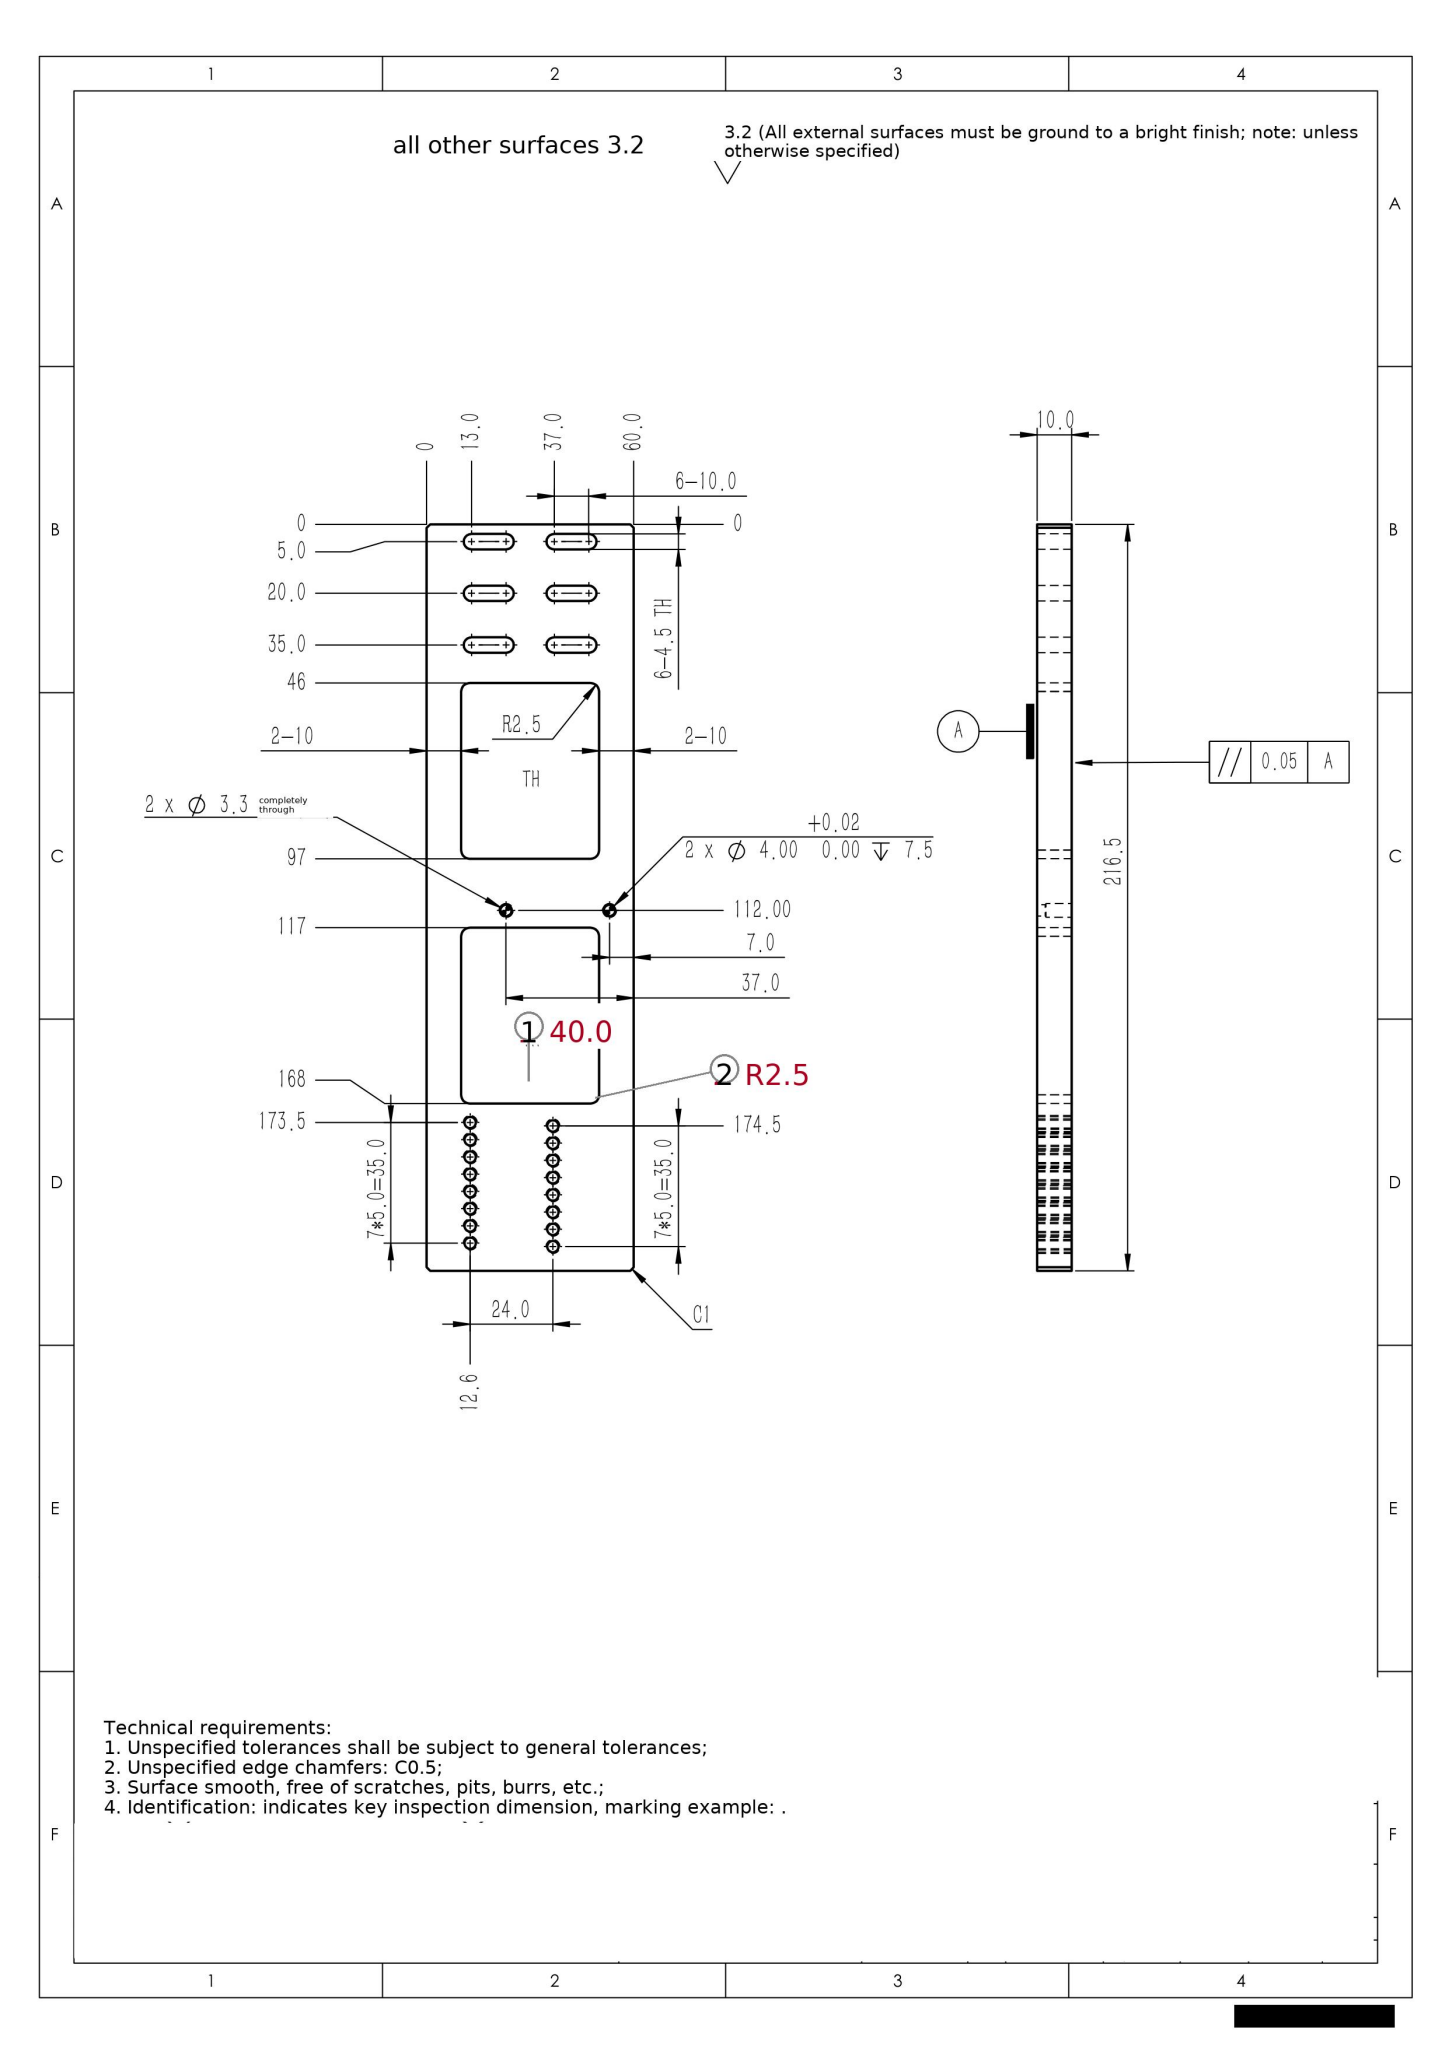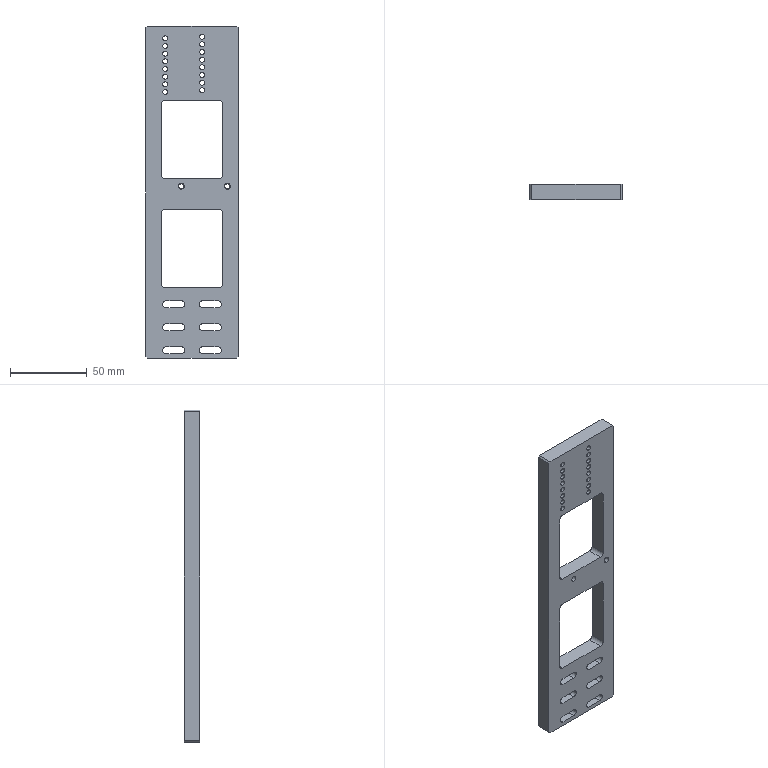Part | SolidWorks | mm | 1 solid | 94 faces | box 60 x 10 x 216.5 mm | volume 83932 mm3 | cylinder 60 | plane 30 | cone 4 | commonest cylinder face diameters 3.3 x36 4.5 x12 5 x8 4 x4
build123d program:
from build123d import *

# Parameters (mm, degrees)
SKETCH1_W                     = 60
SKETCH1_H                     = 216.5
BOSS_EXTRUDE1_DEPTH           = 5
CUT_EXTRUDE2_DEPTH            = 113.774
SKETCH9_W                     = 40
SKETCH9_H                     = 51
CUT_EXTRUDE5_DEPTH            = 113.774
FILLET1_R                     = 2.5
M4_TAPPED_HOLE1_D             = 3.3
SIZE_MM_DOWEL_PIN_HOLE1_D     = 4
SIZE_MM_DOWEL_PIN_HOLE1_DEPTH = 7.5
SIZE_MM_DOWEL_PIN_HOLE1_TIP   = 1.202
F_3_3_3_3_DIAMETER_HOLE1_D    = 3.3
CHAMFER1_SIZE                 = 1


with BuildPart() as part:
    # Sketch1 → Boss-Extrude1 (new, symmetric)
    with BuildSketch(Plane(origin=(0, 0, 0), x_dir=(1, 0, 0), z_dir=(0, 1, 0))):
        Rectangle(SKETCH1_W, SKETCH1_H)
    extrude(amount=BOSS_EXTRUDE1_DEPTH, both=True)

    # Sketch6 → Cut-Extrude2 (cut, through all)
    with BuildSketch(Plane(origin=(0, 5, 0), x_dir=(1, 0, 0), z_dir=(0, 1, 0))):
        with BuildLine():
            Line((-17, 105.5), (-7, 105.5))
            ThreePointArc((-7, 105.5), (-4.75, 103.25), (-7, 101))
            Line((-7, 101), (-17, 101))
            ThreePointArc((-17, 101), (-19.25, 103.25), (-17, 105.5))
        make_face()
        with BuildLine():
            Line((7, 105.5), (17, 105.5))
            ThreePointArc((17, 105.5), (19.25, 103.25), (17, 101))
            Line((17, 101), (7, 101))
            ThreePointArc((7, 101), (4.75, 103.25), (7, 105.5))
        make_face()
        with BuildLine():
            Line((-17, 90.5), (-7, 90.5))
            ThreePointArc((-7, 90.5), (-4.75, 88.25), (-7, 86))
            Line((-7, 86), (-17, 86))
            ThreePointArc((-17, 86), (-19.25, 88.25), (-17, 90.5))
        make_face()
        with BuildLine():
            Line((7, 90.5), (17, 90.5))
            ThreePointArc((17, 90.5), (19.25, 88.25), (17, 86))
            Line((17, 86), (7, 86))
            ThreePointArc((7, 86), (4.75, 88.25), (7, 90.5))
        make_face()
        with BuildLine():
            Line((-17, 75.5), (-7, 75.5))
            ThreePointArc((-7, 75.5), (-4.75, 73.25), (-7, 71))
            Line((-7, 71), (-17, 71))
            ThreePointArc((-17, 71), (-19.25, 73.25), (-17, 75.5))
        make_face()
        with BuildLine():
            Line((7, 75.5), (17, 75.5))
            ThreePointArc((17, 75.5), (19.25, 73.25), (17, 71))
            Line((17, 71), (7, 71))
            ThreePointArc((7, 71), (4.75, 73.25), (7, 75.5))
        make_face()
    extrude(amount=-CUT_EXTRUDE2_DEPTH, mode=Mode.SUBTRACT)

    # Sketch9 → Cut-Extrude5 (cut, through all)
    with BuildSketch(Plane(origin=(0, 5, 0), x_dir=(1, 0, 0), z_dir=(0, 1, 0))):
        with Locations((0, 36.75)):
            Rectangle(SKETCH9_W, SKETCH9_H)
        with Locations((0, -34.25)):
            Rectangle(SKETCH9_W, SKETCH9_H)
    extrude(amount=-CUT_EXTRUDE5_DEPTH, mode=Mode.SUBTRACT)

    # Fillet1
    fillet1_edges = [part.edges().sort_by_distance(p)[0] for p in [
        (-20, 0, -11.25),
        (-20, 0, -62.25),
        (20, 0, -62.25),
        (20, 0, -11.25),
        (-20, 0, 59.75),
        (-20, 0, 8.75),
        (20, 0, 8.75),
        (20, 0, 59.75),
    ]]
    fillet(fillet1_edges, radius=FILLET1_R)

    # M4 Tapped Hole1 (through all)
    with Locations(Plane(origin=(0, 5, 0), x_dir=(1, 0, 0), z_dir=(0, 1, 0))):
        with Locations((-17.4, -75.25), (-17.4, -80.25), (-17.4, -85.25), (-17.4, -90.25), (-17.4, -95.25), (-17.4, -100.25), (6.58, -76.25), (6.58, -81.25), (6.58, -86.25), (6.58, -91.25), (6.58, -96.25), (6.58, -101.25), (-17.4, -70.25), (6.58, -71.25), (6.58, -66.25), (-17.4, -65.25)):
            Hole(M4_TAPPED_HOLE1_D / 2)

    # Size mm Dowel Pin Hole1
    with Locations(Plane(origin=(0, -5, 0), x_dir=(-1, 0, 0), z_dir=(0, -1, 0))):
        with Locations((-23, -3.75), (7, -3.75)):
            Hole(SIZE_MM_DOWEL_PIN_HOLE1_D / 2, depth=SIZE_MM_DOWEL_PIN_HOLE1_DEPTH)
            with Locations((0, 0, -(SIZE_MM_DOWEL_PIN_HOLE1_DEPTH + SIZE_MM_DOWEL_PIN_HOLE1_TIP / 2))):  # 118° drill point
                Cone(0, SIZE_MM_DOWEL_PIN_HOLE1_D / 2, SIZE_MM_DOWEL_PIN_HOLE1_TIP, mode=Mode.SUBTRACT)

    # 3.3 _3.3_ Diameter Hole1 (through all)
    with Locations(Plane(origin=(0, -5, 0), x_dir=(-1, 0, 0), z_dir=(0, -1, 0))):
        with Locations((-23, -3.75), (7, -3.75)):
            Hole(F_3_3_3_3_DIAMETER_HOLE1_D / 2)

    # Chamfer1
    chamfer1_edges = [part.edges().sort_by_distance(p)[0] for p in [
        (30, 0, 108.25),
        (-30, 0, 108.25),
        (-30, 0, -108.25),
        (30, 0, -108.25),
    ]]
    chamfer(chamfer1_edges, length=CHAMFER1_SIZE)


solid = part.part